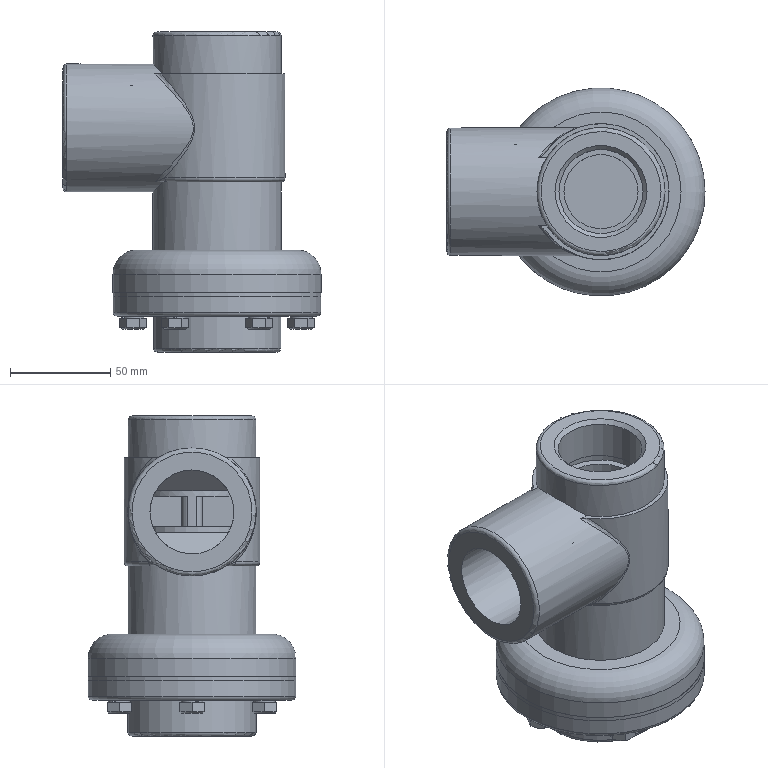Assembly | NX | mm | 28 component files | 28 solids | 476 faces | box 129 x 104 x 160 mm | volume 578680 mm3 | plane 273 | cylinder 126 | cone 37 | spline 34 | torus 6 | commonest cylinder face diameters 42 x15 9 x12 8 x11 11 x10 30 x9 5 x8 7.785 x6 7.9 x6
Bill of materials:
unnamed part 1 | 1 |  | Flat circular disc with a large central bore, four small through-holes evenly spaced on a bolt circle, and short rectangular lugs projecting from the underside.
unnamed part 2 | 1 |  | Short cylindrical cup: thick-walled cylinder with a concentric recess open at one end.
unnamed part 3 | 1 |  | Thin planar loop of round-section wire bent into an octagon-like outline (straight sides with chamfered or rounded corners), with one small gap.
unnamed part 4 | 1 |  | Flanged bushing-like part: circular flange with a central through-bore and six through-holes on a bolt circle, plus a concentric cylindrical boss on one side.
unnamed part 5 | 6 |  | Hex-head bolt-like part: hexagonal head with chamfered corners on the bearing side, and a plain cylindrical shank with a chamfered end.
unnamed part 6 | 4 |  | Flat split washer-like ring: annulus of rectangular section with one narrow angled radial slot.
unnamed part 7 | 1 |  | Helical coil spring of round wire with a uniform diameter and many closely spaced coils, with a flat end face at one end.
unnamed part 8 | 1 |  | Thin flat annular plate or gasket-like ring with a large central opening and six through-holes evenly spaced on a bolt circle.
unnamed part 9 | 1 |  | Cylindrical body with a slotted, reduced-diameter upper section capped by a chamfered disc head, resembling a snap-fit plug or cap.
unnamed part 10 | 6 |  | Split ring of rectangular section with one angled gap, resembling a spring-type lock washer.
unnamed part 11 | 1 |  | Branch (tee-like) fitting: vertical cylindrical body with a through-bore, a rounded base flange, a raised collar band, and a lateral cylindrical branch joining the upper body.
unnamed part 12 | 4 |  | Hex-head bolt-like part with a small cross-hole drilled through the head, and a plain cylindrical shank with a chamfered end.
Mates:
1. fix | VALVE_BODY 1 component
2. touch align | VALVE_DISC 1 face | VALVE_BODY 1 face
3. touch align | VALVE_DISC 1 edge | VALVE_BODY 1 edge
4. touch align | SPRING_CYLINDER_COMPRESSION_1 1 datumaxis | VALVE_DISC 1 face
5. touch align | VALVE_DISC 1 face | SPRING_CYLINDER_COMPRESSION_1 1 face
6. concentric | CUP 1 edge | VALVE_DISC 1 edge
7. concentric | COVER 1 arc | VALVE_DISC 1 edge
8. concentric | VALVE_DISC 1 edge | COVER 1 arc
9. concentric | SPRING_WASHER_4 4 arc | COVER 1 edge
10. concentric | SPRING_WASHER_4 4 edge | BOLT_M4_X_10 4 edge
11. fix | assembly component
12. bond | BOLT_M4_X_10 4 component | assembly component
13. bond | SPRING_WASHER_4 4 component | assembly component
14. bond | BOLT_M4_X_10 3 component | assembly component
15. bond | SPRING_WASHER_4 3 component | assembly component
16. bond | BOLT_M4_X_10 2 component | assembly component
17. bond | SPRING_WASHER_4 2 component | assembly component
18. bond | BOLT_M4_X_10 1 component | assembly component
19. bond | SPRING_WASHER_4 1 component | assembly component
20. circular | assembly datumaxis | assembly cartesiancoordinatesystem | assembly cartesiancoordinatesystem | assembly cartesiancoordinatesystem | assembly cartesiancoordinatesystem
21. circular | assembly datumaxis | assembly cartesiancoordinatesystem | assembly cartesiancoordinatesystem | assembly cartesiancoordinatesystem | assembly cartesiancoordinatesystem
22. touch align | STEEL_WIRE 1 line | BOLT_M4_X_10 4 face
23. touch align | STEEL_WIRE 1 line | BOLT_M4_X_10 1 face
24. concentric | WASHER 1 arc | VALVE_BODY 1 edge
25. concentric | WASHER 1 arc | VALVE_BODY 1 edge
26. concentric | WASHER 1 edge | END_CAP 1 edge
27. concentric | END_CAP 1 edge | WASHER 1 edge
28. concentric | SPRING_WASHER 6 arc | END_CAP 1 edge
29. concentric | SPRING_WASHER 6 edge | BOLT_M8_x_20 6 edge
30. fix | assembly component
31. bond | SPRING_WASHER 6 component | assembly component
32. bond | BOLT_M8_x_20 6 component | assembly component
33. bond | SPRING_WASHER 5 component | assembly component
34. bond | BOLT_M8_x_20 5 component | assembly component
35. bond | SPRING_WASHER 4 component | assembly component
36. bond | BOLT_M8_x_20 4 component | assembly component
37. bond | SPRING_WASHER 3 component | assembly component
38. bond | BOLT_M8_x_20 3 component | assembly component
39. bond | SPRING_WASHER 2 component | assembly component
40. bond | BOLT_M8_x_20 2 component | assembly component
41. bond | SPRING_WASHER 1 component | assembly component
42. bond | BOLT_M8_x_20 1 component | assembly component
43. circular | assembly datumaxis | assembly cartesiancoordinatesystem | assembly cartesiancoordinatesystem | assembly cartesiancoordinatesystem | assembly cartesiancoordinatesystem | assembly cartesiancoordinatesystem | assembly cartesiancoordinatesystem
44. circular | assembly datumaxis | assembly cartesiancoordinatesystem | assembly cartesiancoordinatesystem | assembly cartesiancoordinatesystem | assembly cartesiancoordinatesystem | assembly cartesiancoordinatesystem | assembly cartesiancoordinatesystem